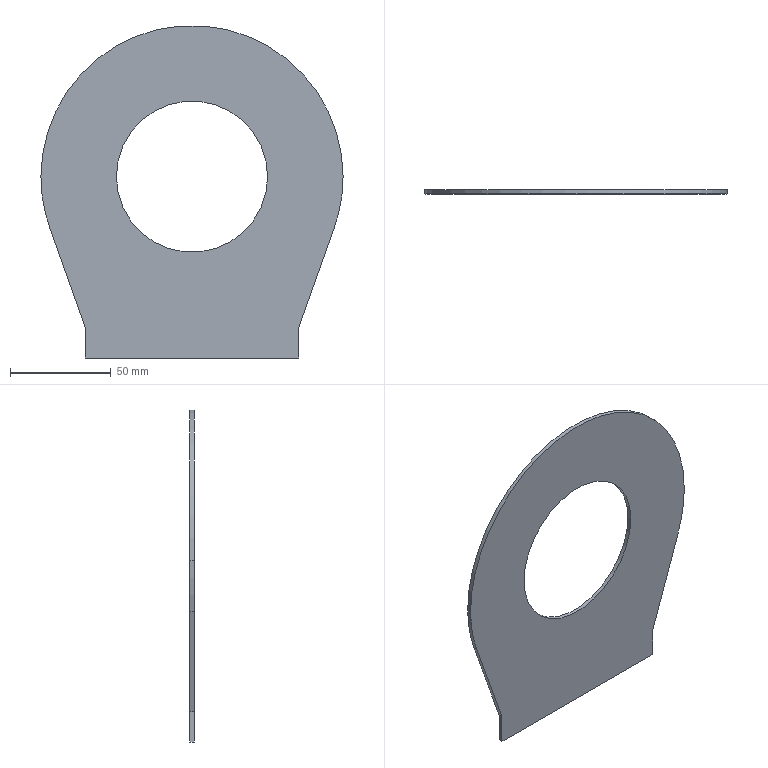Component | SolidWorks | ArmHousing2-1 | 1 solid | 12 faces | box 150 x 2 x 165 mm | volume 31737 mm3 | plane 7 | cylinder 5 | commonest cylinder face diameters 150 x3 75 x2
build123d program:
from build123d import *

# Parameters (mm, degrees)
SKETCH2_R           = 37.5
BOSS_EXTRUDE1_DEPTH = 2


with BuildPart() as part:
    # Sketch2 → Boss-Extrude1 (new body)
    with BuildSketch(Plane(origin=(0, 315.63, 5.509), x_dir=(1, 0, 0), z_dir=(0, 0.9998, 0.01745))):
        with BuildLine():
            Line((15, 168.44), (64.895, 150.716))
            ThreePointArc((64.895, 150.716), (165, 221.39), (64.895, 292.063))
            Line((64.895, 292.063), (15, 274.34))
            Line((15, 274.34), (0, 274.34))
            Line((0, 274.34), (0, 168.44))
            Line((0, 168.44), (15, 168.44))
        make_face()
        with Locations(Location((90, 221.39, 0), (0, 0, 90))):
            Circle(SKETCH2_R, mode=Mode.SUBTRACT)
    extrude(amount=BOSS_EXTRUDE1_DEPTH)


solid = part.part

# Placed as in the assembly
solid = solid.moved(Location((365.049, 644.321, -2182.934), (-90, -89, -90)))
STEP:
#1=COLOUR_RGB('',0.7922,0.8196,0.9333);
#2=FILL_AREA_STYLE_COLOUR('',#1);
#3=FILL_AREA_STYLE('',(#2));
#4=SURFACE_STYLE_FILL_AREA(#3);
#5=SURFACE_SIDE_STYLE('',(#4));
#6=SURFACE_STYLE_USAGE(.BOTH.,#5);
#7=PRESENTATION_STYLE_ASSIGNMENT((#6));
#8=CARTESIAN_POINT('',(24.565,37.874,-82.399));
#9=VERTEX_POINT('',#8);
#10=CARTESIAN_POINT('',(21.612,37.874,-82.399));
#11=VERTEX_POINT('',#10);
#12=CARTESIAN_POINT('',(23.088,37.874,-82.399));
#13=DIRECTION('',(-0.,1.,0.));
#14=DIRECTION('',(-1.,0.,0.));
#15=AXIS2_PLACEMENT_3D('',#12,#13,#14);
#16=CIRCLE('',#15,1.476);
#17=EDGE_CURVE('',#9,#11,#16,.T.);
#18=ORIENTED_EDGE('',*,*,#17,.T.);
#19=CARTESIAN_POINT('',(21.612,37.795,-82.399));
#20=VERTEX_POINT('',#19);
#21=CARTESIAN_POINT('',(21.612,37.874,-82.399));
#22=DIRECTION('',(0.,-1.,-0.));
#23=VECTOR('',#22,39.37);
#24=LINE('',#21,#23);
#25=EDGE_CURVE('',#11,#20,#24,.T.);
#26=ORIENTED_EDGE('',*,*,#25,.T.);
#27=CARTESIAN_POINT('',(24.565,37.795,-82.399));
#28=VERTEX_POINT('',#27);
#29=CARTESIAN_POINT('',(23.088,37.795,-82.399));
#30=DIRECTION('',(-0.,1.,0.));
#31=DIRECTION('',(-1.,0.,0.));
#32=AXIS2_PLACEMENT_3D('',#29,#30,#31);
#33=CIRCLE('',#32,1.476);
#34=EDGE_CURVE('',#28,#20,#33,.T.);
#35=ORIENTED_EDGE('',*,*,#34,.F.);
#36=CARTESIAN_POINT('',(24.565,37.874,-82.399));
#37=DIRECTION('',(0.,-1.,-0.));
#38=VECTOR('',#37,39.37);
#39=LINE('',#36,#38);
#40=EDGE_CURVE('',#9,#28,#39,.T.);
#41=ORIENTED_EDGE('',*,*,#40,.F.);
#42=EDGE_LOOP('',(#18,#26,#35,#41));
#43=FACE_OUTER_BOUND('',#42,.T.);
#44=CARTESIAN_POINT('',(23.088,37.874,-82.399));
#45=DIRECTION('',(0.,-1.,-0.));
#46=DIRECTION('',(1.,0.,0.));
#47=AXIS2_PLACEMENT_3D('',#44,#45,#46);
#48=CYLINDRICAL_SURFACE('',#47,1.476);
#49=ADVANCED_FACE('',(#43),#48,.F.);
#50=CARTESIAN_POINT('',(20.135,37.874,-82.399));
#51=VERTEX_POINT('',#50);
#52=CARTESIAN_POINT('',(26.041,37.874,-82.399));
#53=VERTEX_POINT('',#52);
#54=CARTESIAN_POINT('',(23.088,37.874,-82.399));
#55=DIRECTION('',(-0.,1.,0.));
#56=DIRECTION('',(-1.,0.,0.));
#57=AXIS2_PLACEMENT_3D('',#54,#55,#56);
#58=CIRCLE('',#57,2.953);
#59=EDGE_CURVE('',#51,#53,#58,.T.);
#60=ORIENTED_EDGE('',*,*,#59,.F.);
#61=CARTESIAN_POINT('',(20.135,37.795,-82.399));
#62=VERTEX_POINT('',#61);
#63=CARTESIAN_POINT('',(20.135,37.874,-82.399));
#64=DIRECTION('',(0.,-1.,-0.));
#65=VECTOR('',#64,39.37);
#66=LINE('',#63,#65);
#67=EDGE_CURVE('',#51,#62,#66,.T.);
#68=ORIENTED_EDGE('',*,*,#67,.T.);
#69=CARTESIAN_POINT('',(26.041,37.795,-82.399));
#70=VERTEX_POINT('',#69);
#71=CARTESIAN_POINT('',(23.088,37.795,-82.399));
#72=DIRECTION('',(-0.,1.,0.));
#73=DIRECTION('',(-1.,0.,0.));
#74=AXIS2_PLACEMENT_3D('',#71,#72,#73);
#75=CIRCLE('',#74,2.953);
#76=EDGE_CURVE('',#62,#70,#75,.T.);
#77=ORIENTED_EDGE('',*,*,#76,.T.);
#78=CARTESIAN_POINT('',(26.041,37.874,-82.399));
#79=DIRECTION('',(0.,-1.,-0.));
#80=VECTOR('',#79,39.37);
#81=LINE('',#78,#80);
#82=EDGE_CURVE('',#53,#70,#81,.T.);
#83=ORIENTED_EDGE('',*,*,#82,.F.);
#84=EDGE_LOOP('',(#60,#68,#77,#83));
#85=FACE_OUTER_BOUND('',#84,.T.);
#86=CARTESIAN_POINT('',(23.088,37.874,-82.399));
#87=DIRECTION('',(0.,-1.,-0.));
#88=DIRECTION('',(1.,0.,0.));
#89=AXIS2_PLACEMENT_3D('',#86,#87,#88);
#90=CYLINDRICAL_SURFACE('',#89,2.953);
#91=ADVANCED_FACE('',(#85),#90,.T.);
#92=CARTESIAN_POINT('',(25.871,37.874,-83.387));
#93=VERTEX_POINT('',#92);
#94=CARTESIAN_POINT('',(23.088,37.874,-82.399));
#95=DIRECTION('',(-0.,1.,0.));
#96=DIRECTION('',(-1.,0.,0.));
#97=AXIS2_PLACEMENT_3D('',#94,#95,#96);
#98=CIRCLE('',#97,2.953);
#99=EDGE_CURVE('',#53,#93,#98,.T.);
#100=ORIENTED_EDGE('',*,*,#99,.F.);
#101=ORIENTED_EDGE('',*,*,#82,.T.);
#102=CARTESIAN_POINT('',(25.871,37.795,-83.387));
#103=VERTEX_POINT('',#102);
#104=CARTESIAN_POINT('',(23.088,37.795,-82.399));
#105=DIRECTION('',(-0.,1.,0.));
#106=DIRECTION('',(-1.,0.,0.));
#107=AXIS2_PLACEMENT_3D('',#104,#105,#106);
#108=CIRCLE('',#107,2.953);
#109=EDGE_CURVE('',#70,#103,#108,.T.);
#110=ORIENTED_EDGE('',*,*,#109,.T.);
#111=CARTESIAN_POINT('',(25.871,37.874,-83.387));
#112=DIRECTION('',(0.,-1.,-0.));
#113=VECTOR('',#112,39.37);
#114=LINE('',#111,#113);
#115=EDGE_CURVE('',#93,#103,#114,.T.);
#116=ORIENTED_EDGE('',*,*,#115,.F.);
#117=EDGE_LOOP('',(#100,#101,#110,#116));
#118=FACE_OUTER_BOUND('',#117,.T.);
#119=CARTESIAN_POINT('',(23.088,37.874,-82.399));
#120=DIRECTION('',(0.,-1.,-0.));
#121=DIRECTION('',(1.,0.,0.));
#122=AXIS2_PLACEMENT_3D('',#119,#120,#121);
#123=CYLINDRICAL_SURFACE('',#122,2.953);
#124=ADVANCED_FACE('',(#118),#123,.T.);
#125=CARTESIAN_POINT('',(21.003,37.874,-85.942));
#126=VERTEX_POINT('',#125);
#127=CARTESIAN_POINT('',(21.003,37.874,-85.352));
#128=VERTEX_POINT('',#127);
#129=CARTESIAN_POINT('',(21.003,37.874,-85.942));
#130=DIRECTION('',(0.,-0.,1.));
#131=VECTOR('',#130,39.37);
#132=LINE('',#129,#131);
#133=EDGE_CURVE('',#126,#128,#132,.T.);
#134=ORIENTED_EDGE('',*,*,#133,.T.);
#135=CARTESIAN_POINT('',(20.306,37.874,-83.387));
#136=VERTEX_POINT('',#135);
#137=CARTESIAN_POINT('',(21.003,37.874,-85.352));
#138=DIRECTION('',(-0.3347,-0.,0.9423));
#139=VECTOR('',#138,39.37);
#140=LINE('',#137,#139);
#141=EDGE_CURVE('',#128,#136,#140,.T.);
#142=ORIENTED_EDGE('',*,*,#141,.T.);
#143=CARTESIAN_POINT('',(23.088,37.874,-82.399));
#144=DIRECTION('',(-0.,1.,0.));
#145=DIRECTION('',(-1.,0.,0.));
#146=AXIS2_PLACEMENT_3D('',#143,#144,#145);
#147=CIRCLE('',#146,2.953);
#148=EDGE_CURVE('',#136,#51,#147,.T.);
#149=ORIENTED_EDGE('',*,*,#148,.T.);
#150=ORIENTED_EDGE('',*,*,#59,.T.);
#151=ORIENTED_EDGE('',*,*,#99,.T.);
#152=CARTESIAN_POINT('',(25.173,37.874,-85.352));
#153=VERTEX_POINT('',#152);
#154=CARTESIAN_POINT('',(25.871,37.874,-83.387));
#155=DIRECTION('',(-0.3347,0.,-0.9423));
#156=VECTOR('',#155,39.37);
#157=LINE('',#154,#156);
#158=EDGE_CURVE('',#93,#153,#157,.T.);
#159=ORIENTED_EDGE('',*,*,#158,.T.);
#160=CARTESIAN_POINT('',(25.173,37.874,-85.942));
#161=VERTEX_POINT('',#160);
#162=CARTESIAN_POINT('',(25.173,37.874,-85.352));
#163=DIRECTION('',(-0.,0.,-1.));
#164=VECTOR('',#163,39.37);
#165=LINE('',#162,#164);
#166=EDGE_CURVE('',#153,#161,#165,.T.);
#167=ORIENTED_EDGE('',*,*,#166,.T.);
#168=CARTESIAN_POINT('',(25.173,37.874,-85.942));
#169=DIRECTION('',(-1.,0.,0.));
#170=VECTOR('',#169,39.37);
#171=LINE('',#168,#170);
#172=EDGE_CURVE('',#161,#126,#171,.T.);
#173=ORIENTED_EDGE('',*,*,#172,.T.);
#174=EDGE_LOOP('',(#134,#142,#149,#150,#151,#159,#167,#173));
#175=FACE_OUTER_BOUND('',#174,.T.);
#176=ORIENTED_EDGE('',*,*,#17,.F.);
#177=CARTESIAN_POINT('',(23.088,37.874,-82.399));
#178=DIRECTION('',(-0.,1.,0.));
#179=DIRECTION('',(-1.,0.,0.));
#180=AXIS2_PLACEMENT_3D('',#177,#178,#179);
#181=CIRCLE('',#180,1.476);
#182=EDGE_CURVE('',#11,#9,#181,.T.);
#183=ORIENTED_EDGE('',*,*,#182,.F.);
#184=EDGE_LOOP('',(#176,#183));
#185=FACE_BOUND('',#184,.T.);
#186=CARTESIAN_POINT('',(23.088,37.874,-82.399));
#187=DIRECTION('',(-0.,1.,0.));
#188=DIRECTION('',(-1.,-0.,0.));
#189=AXIS2_PLACEMENT_3D('',#186,#187,#188);
#190=PLANE('',#189);
#191=ADVANCED_FACE('',(#175,#185),#190,.T.);
#192=CARTESIAN_POINT('',(21.003,37.795,-85.942));
#193=VERTEX_POINT('',#192);
#194=CARTESIAN_POINT('',(21.003,37.795,-85.352));
#195=VERTEX_POINT('',#194);
#196=CARTESIAN_POINT('',(21.003,37.795,-85.942));
#197=DIRECTION('',(0.,-0.,1.));
#198=VECTOR('',#197,39.37);
#199=LINE('',#196,#198);
#200=EDGE_CURVE('',#193,#195,#199,.T.);
#201=ORIENTED_EDGE('',*,*,#200,.F.);
#202=CARTESIAN_POINT('',(25.173,37.795,-85.942));
#203=VERTEX_POINT('',#202);
#204=CARTESIAN_POINT('',(25.173,37.795,-85.942));
#205=DIRECTION('',(-1.,0.,0.));
#206=VECTOR('',#205,39.37);
#207=LINE('',#204,#206);
#208=EDGE_CURVE('',#203,#193,#207,.T.);
#209=ORIENTED_EDGE('',*,*,#208,.F.);
#210=CARTESIAN_POINT('',(25.173,37.795,-85.352));
#211=VERTEX_POINT('',#210);
#212=CARTESIAN_POINT('',(25.173,37.795,-85.352));
#213=DIRECTION('',(-0.,0.,-1.));
#214=VECTOR('',#213,39.37);
#215=LINE('',#212,#214);
#216=EDGE_CURVE('',#211,#203,#215,.T.);
#217=ORIENTED_EDGE('',*,*,#216,.F.);
#218=CARTESIAN_POINT('',(25.871,37.795,-83.387));
#219=DIRECTION('',(-0.3347,0.,-0.9423));
#220=VECTOR('',#219,39.37);
#221=LINE('',#218,#220);
#222=EDGE_CURVE('',#103,#211,#221,.T.);
#223=ORIENTED_EDGE('',*,*,#222,.F.);
#224=ORIENTED_EDGE('',*,*,#109,.F.);
#225=ORIENTED_EDGE('',*,*,#76,.F.);
#226=CARTESIAN_POINT('',(20.306,37.795,-83.387));
#227=VERTEX_POINT('',#226);
#228=CARTESIAN_POINT('',(23.088,37.795,-82.399));
#229=DIRECTION('',(-0.,1.,0.));
#230=DIRECTION('',(-1.,0.,0.));
#231=AXIS2_PLACEMENT_3D('',#228,#229,#230);
#232=CIRCLE('',#231,2.953);
#233=EDGE_CURVE('',#227,#62,#232,.T.);
#234=ORIENTED_EDGE('',*,*,#233,.F.);
#235=CARTESIAN_POINT('',(21.003,37.795,-85.352));
#236=DIRECTION('',(-0.3347,-0.,0.9423));
#237=VECTOR('',#236,39.37);
#238=LINE('',#235,#237);
#239=EDGE_CURVE('',#195,#227,#238,.T.);
#240=ORIENTED_EDGE('',*,*,#239,.F.);
#241=EDGE_LOOP('',(#201,#209,#217,#223,#224,#225,#234,#240));
#242=FACE_OUTER_BOUND('',#241,.T.);
#243=ORIENTED_EDGE('',*,*,#34,.T.);
#244=CARTESIAN_POINT('',(23.088,37.795,-82.399));
#245=DIRECTION('',(-0.,1.,0.));
#246=DIRECTION('',(-1.,0.,0.));
#247=AXIS2_PLACEMENT_3D('',#244,#245,#246);
#248=CIRCLE('',#247,1.476);
#249=EDGE_CURVE('',#20,#28,#248,.T.);
#250=ORIENTED_EDGE('',*,*,#249,.T.);
#251=EDGE_LOOP('',(#243,#250));
#252=FACE_BOUND('',#251,.T.);
#253=CARTESIAN_POINT('',(23.088,37.795,-82.399));
#254=DIRECTION('',(-0.,1.,0.));
#255=DIRECTION('',(-1.,-0.,0.));
#256=AXIS2_PLACEMENT_3D('',#253,#254,#255);
#257=PLANE('',#256);
#258=ADVANCED_FACE('',(#242,#252),#257,.F.);
#259=ORIENTED_EDGE('',*,*,#200,.T.);
#260=CARTESIAN_POINT('',(21.003,37.874,-85.352));
#261=DIRECTION('',(0.,-1.,-0.));
#262=VECTOR('',#261,39.37);
#263=LINE('',#260,#262);
#264=EDGE_CURVE('',#128,#195,#263,.T.);
#265=ORIENTED_EDGE('',*,*,#264,.F.);
#266=ORIENTED_EDGE('',*,*,#133,.F.);
#267=CARTESIAN_POINT('',(21.003,37.874,-85.942));
#268=DIRECTION('',(0.,-1.,-0.));
#269=VECTOR('',#268,39.37);
#270=LINE('',#267,#269);
#271=EDGE_CURVE('',#126,#193,#270,.T.);
#272=ORIENTED_EDGE('',*,*,#271,.T.);
#273=EDGE_LOOP('',(#259,#265,#266,#272));
#274=FACE_OUTER_BOUND('',#273,.T.);
#275=CARTESIAN_POINT('',(21.003,37.874,-85.942));
#276=DIRECTION('',(1.,0.,-0.));
#277=DIRECTION('',(-0.,1.,0.));
#278=AXIS2_PLACEMENT_3D('',#275,#276,#277);
#279=PLANE('',#278);
#280=ADVANCED_FACE('',(#274),#279,.F.);
#281=ORIENTED_EDGE('',*,*,#239,.T.);
#282=CARTESIAN_POINT('',(20.306,37.874,-83.387));
#283=DIRECTION('',(0.,-1.,-0.));
#284=VECTOR('',#283,39.37);
#285=LINE('',#282,#284);
#286=EDGE_CURVE('',#136,#227,#285,.T.);
#287=ORIENTED_EDGE('',*,*,#286,.F.);
#288=ORIENTED_EDGE('',*,*,#141,.F.);
#289=ORIENTED_EDGE('',*,*,#264,.T.);
#290=EDGE_LOOP('',(#281,#287,#288,#289));
#291=FACE_OUTER_BOUND('',#290,.T.);
#292=CARTESIAN_POINT('',(21.003,37.874,-85.352));
#293=DIRECTION('',(0.9423,-0.,0.3347));
#294=DIRECTION('',(0.3347,-0.005843,-0.9423));
#295=AXIS2_PLACEMENT_3D('',#292,#293,#294);
#296=PLANE('',#295);
#297=ADVANCED_FACE('',(#291),#296,.F.);
#298=ORIENTED_EDGE('',*,*,#67,.F.);
#299=ORIENTED_EDGE('',*,*,#148,.F.);
#300=ORIENTED_EDGE('',*,*,#286,.T.);
#301=ORIENTED_EDGE('',*,*,#233,.T.);
#302=EDGE_LOOP('',(#298,#299,#300,#301));
#303=FACE_OUTER_BOUND('',#302,.T.);
#304=CARTESIAN_POINT('',(23.088,37.874,-82.399));
#305=DIRECTION('',(0.,-1.,-0.));
#306=DIRECTION('',(1.,0.,0.));
#307=AXIS2_PLACEMENT_3D('',#304,#305,#306);
#308=CYLINDRICAL_SURFACE('',#307,2.953);
#309=ADVANCED_FACE('',(#303),#308,.T.);
#310=ORIENTED_EDGE('',*,*,#222,.T.);
#311=CARTESIAN_POINT('',(25.173,37.874,-85.352));
#312=DIRECTION('',(0.,-1.,-0.));
#313=VECTOR('',#312,39.37);
#314=LINE('',#311,#313);
#315=EDGE_CURVE('',#153,#211,#314,.T.);
#316=ORIENTED_EDGE('',*,*,#315,.F.);
#317=ORIENTED_EDGE('',*,*,#158,.F.);
#318=ORIENTED_EDGE('',*,*,#115,.T.);
#319=EDGE_LOOP('',(#310,#316,#317,#318));
#320=FACE_OUTER_BOUND('',#319,.T.);
#321=CARTESIAN_POINT('',(25.871,37.874,-83.387));
#322=DIRECTION('',(-0.9423,-0.,0.3347));
#323=DIRECTION('',(0.3347,-0.005843,0.9423));
#324=AXIS2_PLACEMENT_3D('',#321,#322,#323);
#325=PLANE('',#324);
#326=ADVANCED_FACE('',(#320),#325,.F.);
#327=ORIENTED_EDGE('',*,*,#216,.T.);
#328=CARTESIAN_POINT('',(25.173,37.874,-85.942));
#329=DIRECTION('',(0.,-1.,-0.));
#330=VECTOR('',#329,39.37);
#331=LINE('',#328,#330);
#332=EDGE_CURVE('',#161,#203,#331,.T.);
#333=ORIENTED_EDGE('',*,*,#332,.F.);
#334=ORIENTED_EDGE('',*,*,#166,.F.);
#335=ORIENTED_EDGE('',*,*,#315,.T.);
#336=EDGE_LOOP('',(#327,#333,#334,#335));
#337=FACE_OUTER_BOUND('',#336,.T.);
#338=CARTESIAN_POINT('',(25.173,37.874,-85.352));
#339=DIRECTION('',(-1.,-0.,0.));
#340=DIRECTION('',(0.,-1.,-0.));
#341=AXIS2_PLACEMENT_3D('',#338,#339,#340);
#342=PLANE('',#341);
#343=ADVANCED_FACE('',(#337),#342,.F.);
#344=ORIENTED_EDGE('',*,*,#208,.T.);
#345=ORIENTED_EDGE('',*,*,#271,.F.);
#346=ORIENTED_EDGE('',*,*,#172,.F.);
#347=ORIENTED_EDGE('',*,*,#332,.T.);
#348=EDGE_LOOP('',(#344,#345,#346,#347));
#349=FACE_OUTER_BOUND('',#348,.T.);
#350=CARTESIAN_POINT('',(25.173,37.874,-85.942));
#351=DIRECTION('',(0.,-0.,1.));
#352=DIRECTION('',(0.9998,-0.01745,-0.));
#353=AXIS2_PLACEMENT_3D('',#350,#351,#352);
#354=PLANE('',#353);
#355=ADVANCED_FACE('',(#349),#354,.F.);
#356=ORIENTED_EDGE('',*,*,#25,.F.);
#357=ORIENTED_EDGE('',*,*,#182,.T.);
#358=ORIENTED_EDGE('',*,*,#40,.T.);
#359=ORIENTED_EDGE('',*,*,#249,.F.);
#360=EDGE_LOOP('',(#356,#357,#358,#359));
#361=FACE_OUTER_BOUND('',#360,.T.);
#362=CARTESIAN_POINT('',(23.088,37.874,-82.399));
#363=DIRECTION('',(0.,-1.,-0.));
#364=DIRECTION('',(1.,0.,0.));
#365=AXIS2_PLACEMENT_3D('',#362,#363,#364);
#366=CYLINDRICAL_SURFACE('',#365,1.476);
#367=ADVANCED_FACE('',(#361),#366,.F.);
#368=CLOSED_SHELL('',(#49,#91,#124,#191,#258,#280,#297,#309,#326,#343,#355,#367));
#369=MANIFOLD_SOLID_BREP('',#368);
#370=STYLED_ITEM('',(#7),#369);
#371=(LENGTH_UNIT()NAMED_UNIT(*)SI_UNIT($,.METRE.));
#372=LENGTH_MEASURE_WITH_UNIT(LENGTH_MEASURE(0.0254),#371);
#373=DIMENSIONAL_EXPONENTS(1.,0.,0.,0.,0.,0.,0.);
#374=(CONVERSION_BASED_UNIT('',#372)LENGTH_UNIT()NAMED_UNIT(#373));
#375=UNCERTAINTY_MEASURE_WITH_UNIT(LENGTH_MEASURE(0.00001),#374,'','');
#376=(NAMED_UNIT(*)PLANE_ANGLE_UNIT()SI_UNIT($,.RADIAN.));
#377=(NAMED_UNIT(*)SI_UNIT($,.STERADIAN.)SOLID_ANGLE_UNIT());
#378=(GEOMETRIC_REPRESENTATION_CONTEXT(3)GLOBAL_UNCERTAINTY_ASSIGNED_CONTEXT((#375))GLOBAL_UNIT_ASSIGNED_CONTEXT((#374,#376,#377))REPRESENTATION_CONTEXT('',''));
#379=MECHANICAL_DESIGN_GEOMETRIC_PRESENTATION_REPRESENTATION('',(#370),#378);
#380=CARTESIAN_POINT('',(0.,0.,0.));
#381=DIRECTION('',(0.,0.,1.));
#382=DIRECTION('',(1.,0.,0.));
#383=AXIS2_PLACEMENT_3D('',#380,#381,#382);
#384=(LENGTH_UNIT()NAMED_UNIT(*)SI_UNIT($,.METRE.));
#385=LENGTH_MEASURE_WITH_UNIT(LENGTH_MEASURE(0.0254),#384);
#386=DIMENSIONAL_EXPONENTS(1.,0.,0.,0.,0.,0.,0.);
#387=(CONVERSION_BASED_UNIT('',#385)LENGTH_UNIT()NAMED_UNIT(#386));
#388=UNCERTAINTY_MEASURE_WITH_UNIT(LENGTH_MEASURE(0.00001),#387,'','');
#389=(NAMED_UNIT(*)PLANE_ANGLE_UNIT()SI_UNIT($,.RADIAN.));
#390=(NAMED_UNIT(*)SI_UNIT($,.STERADIAN.)SOLID_ANGLE_UNIT());
#391=(GEOMETRIC_REPRESENTATION_CONTEXT(3)GLOBAL_UNCERTAINTY_ASSIGNED_CONTEXT((#388))GLOBAL_UNIT_ASSIGNED_CONTEXT((#387,#389,#390))REPRESENTATION_CONTEXT('',''));
#392=ADVANCED_BREP_SHAPE_REPRESENTATION('',(#369,#383),#391);
#393=PRESENTATION_LAYER_ASSIGNMENT('','',(#370));